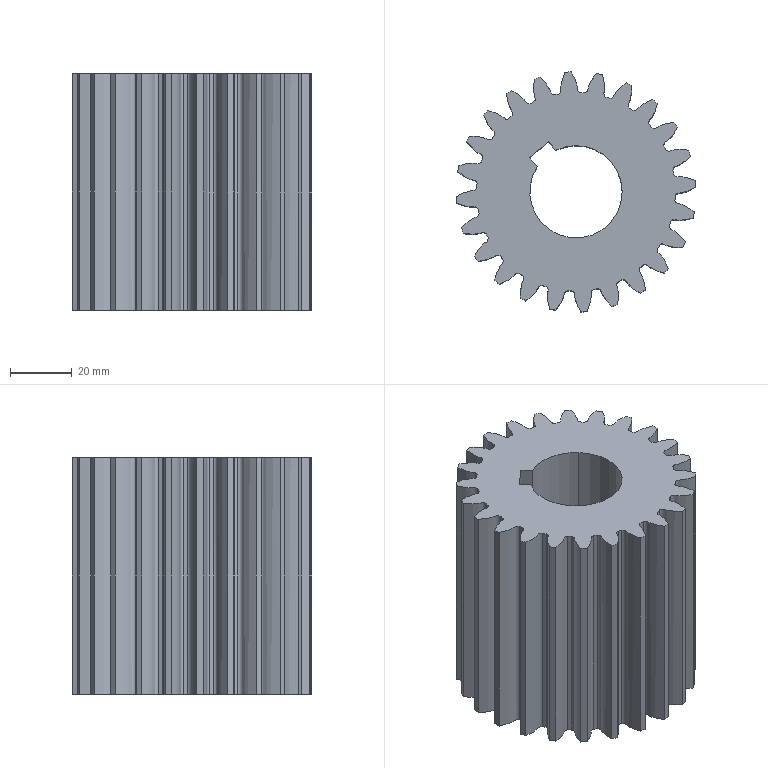Component | SolidWorks | CylindricalGear24_3-1 | 1 solid | 104 faces | volume 250373 mm3 | cylinder 51 | spline 48 | plane 5 | commonest cylinder face diameters 78 x24 64.5 x24 30 x3